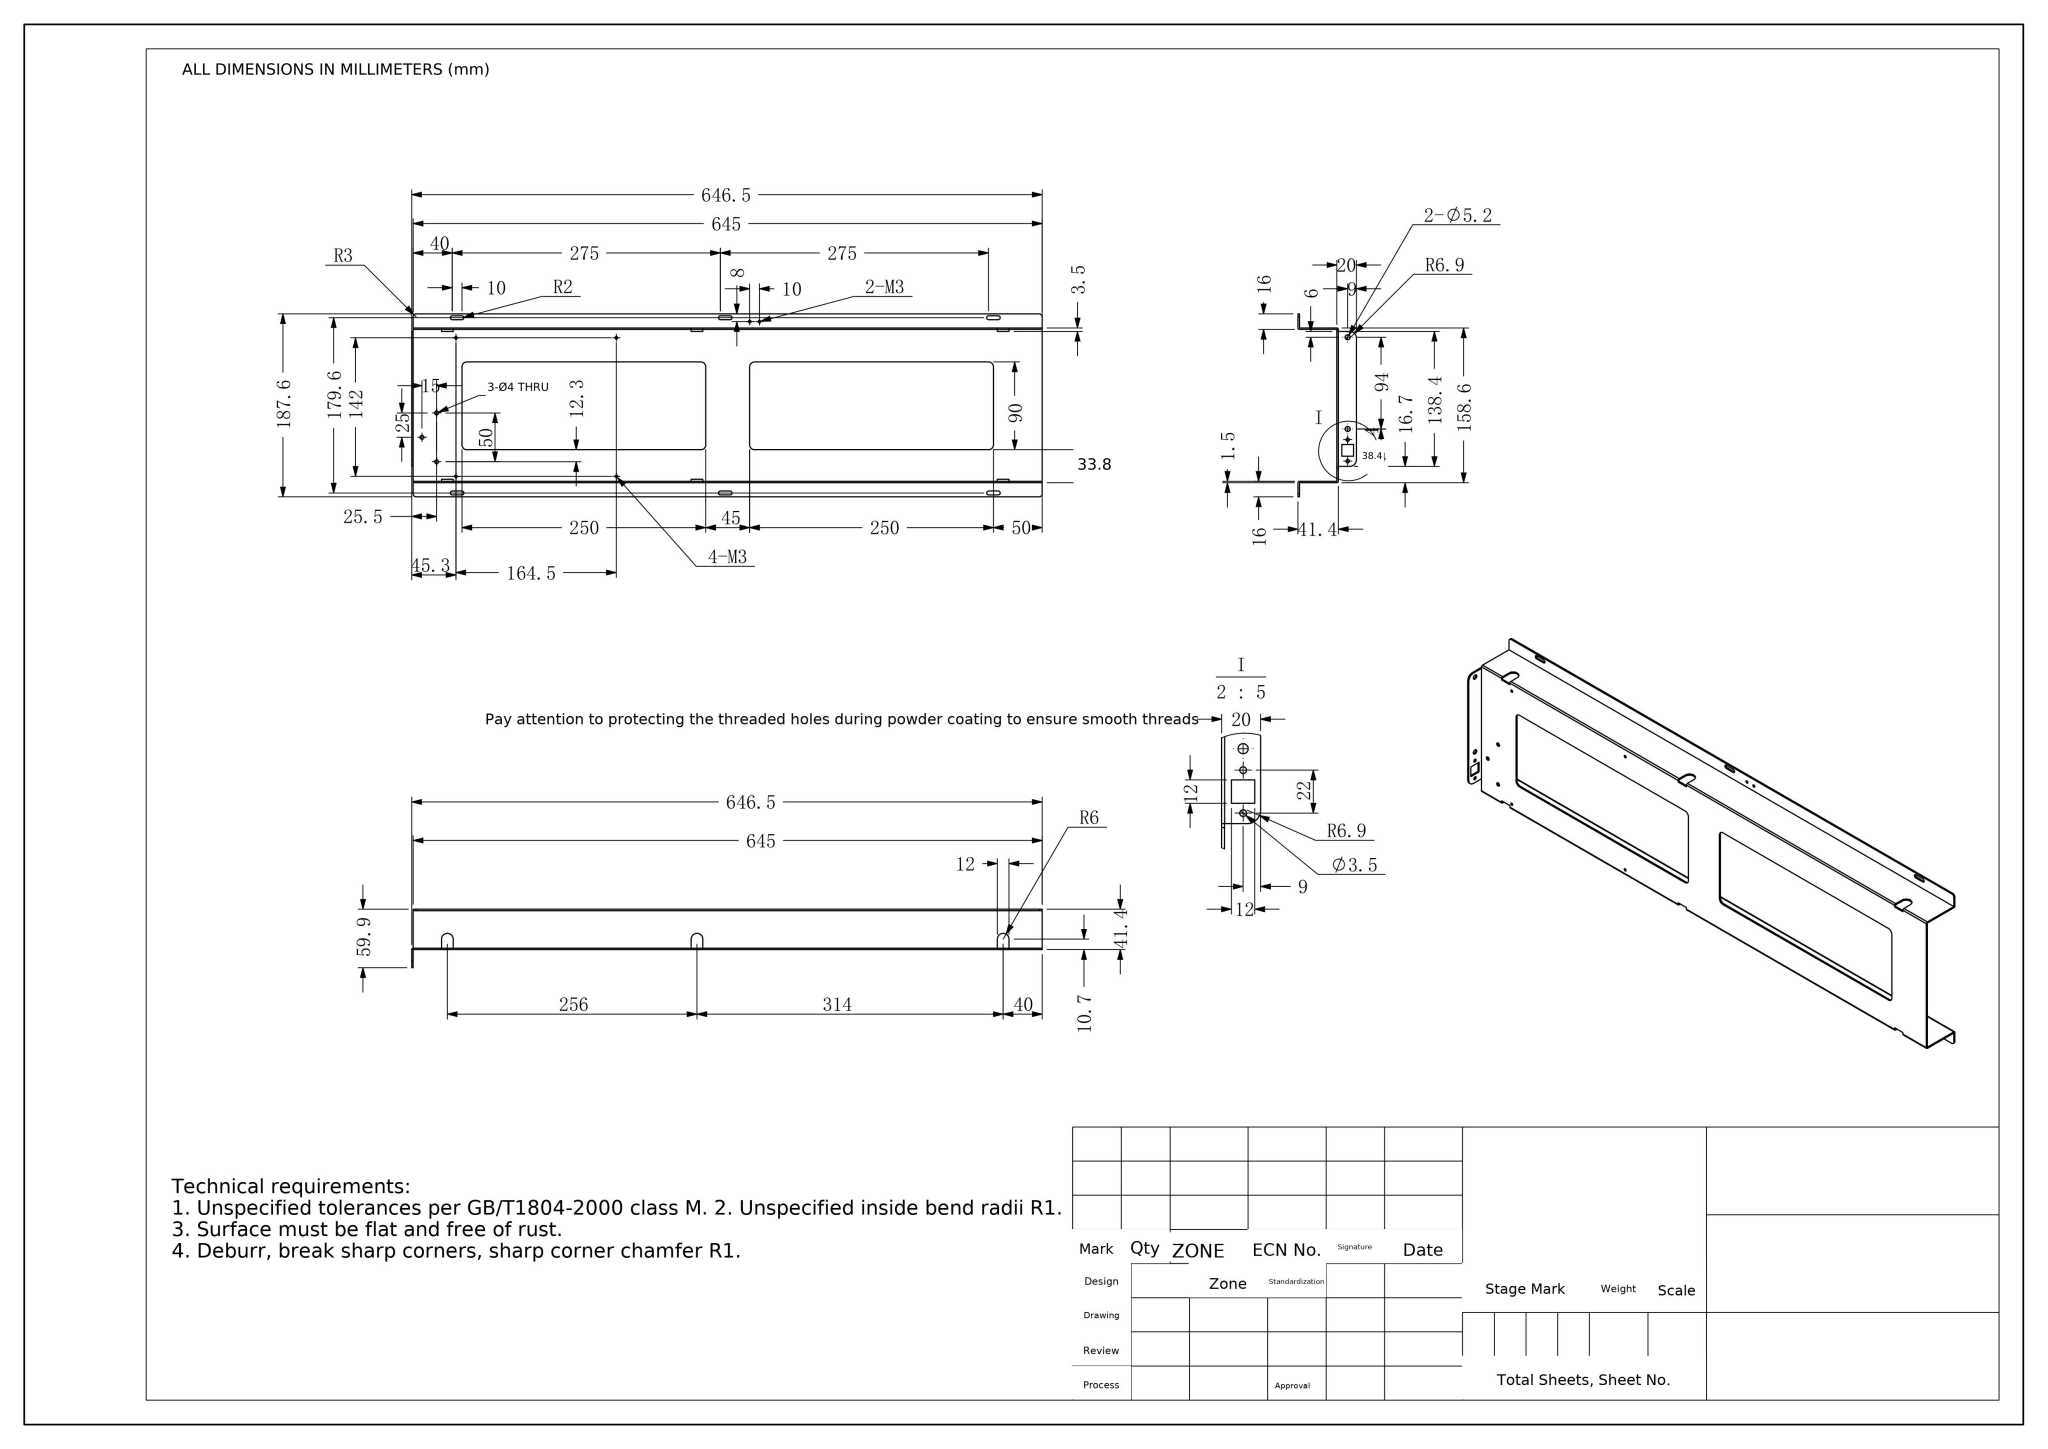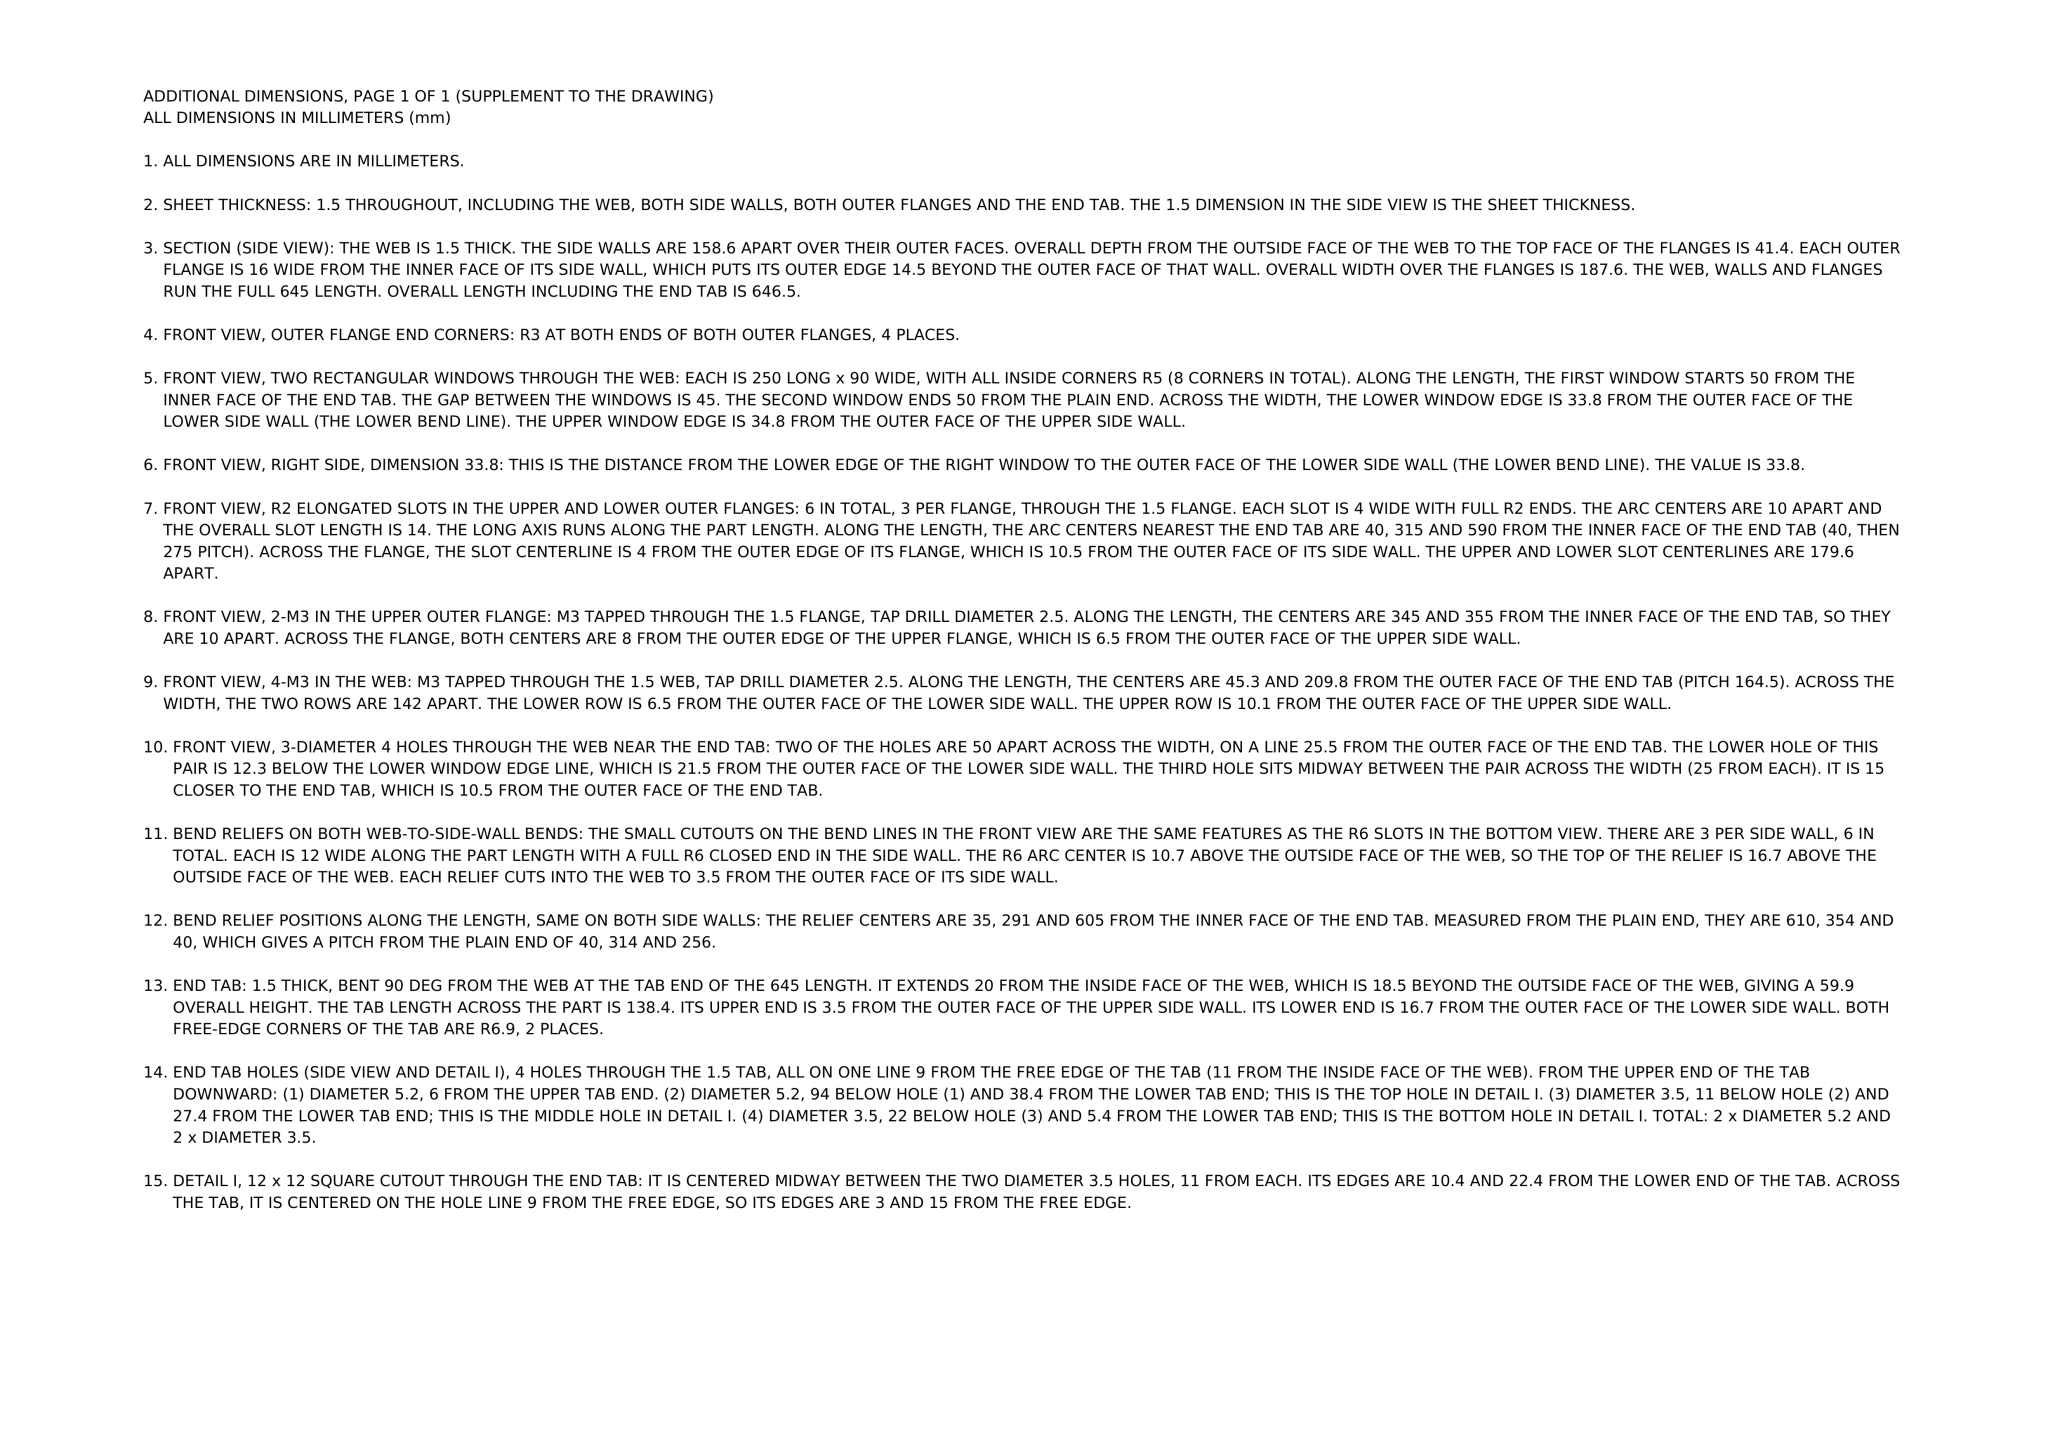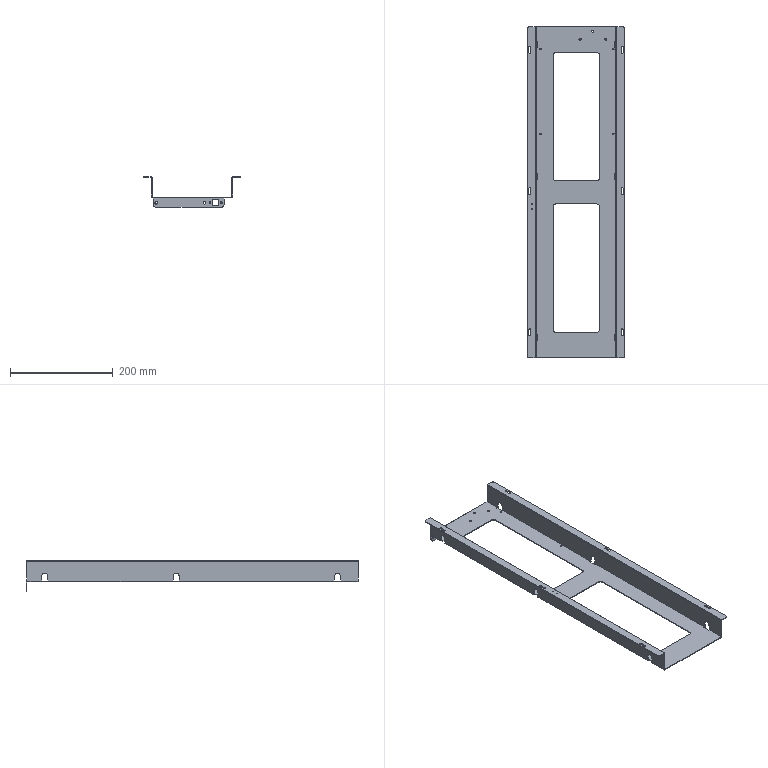Part | NX | mm | 1 solid | 150 faces | box 187.6 x 646.5 x 59.9 mm | volume 191339 mm3 | cylinder 83 | plane 67 | commonest cylinder face diameters 4 x18 2.5 x12 3.004 x11 0.004 x11 12 x9 10 x8 5.2 x4 3.5 x4